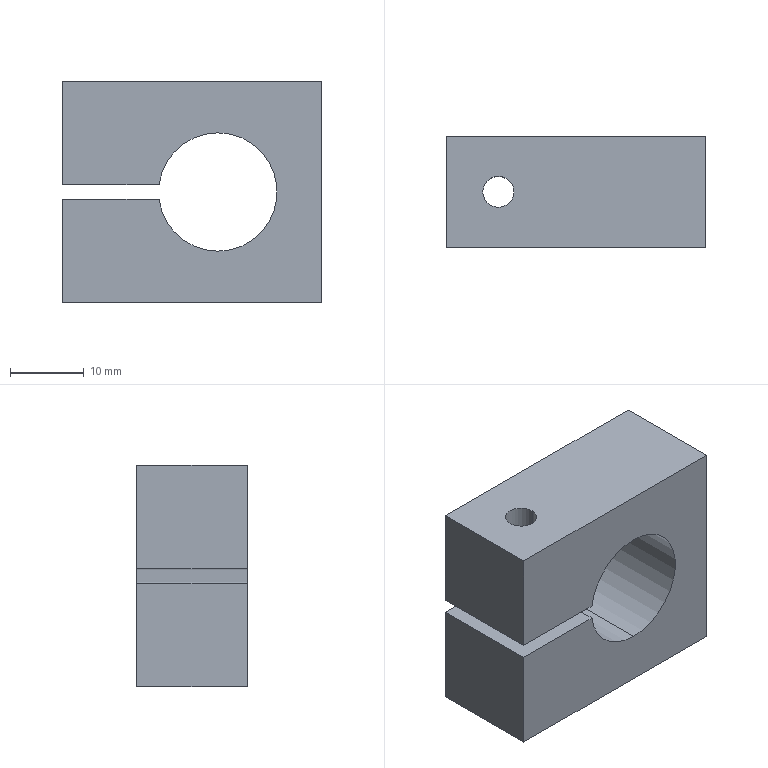Component | SolidWorks | PressingMechanism-11-5 | 1 solid | 19 faces | box 35 x 15 x 30 mm | volume 11521 mm3 | plane 10 | cylinder 9 | commonest cylinder face diameters 16 x3 10 x2 5.5 x2 4.2 x2
build123d program:
from build123d import *

# Parameters (mm, degrees)
SKETCH1_W                                           = 35
SKETCH1_H                                           = 30
EXTRUDE1_DEPTH                                      = 7.5
SKETCH2_R                                           = 8
EXTRUDE2_DEPTH                                      = 28.5
SKETCH3_W                                           = 21
SKETCH3_H                                           = 2
CUT_EXTRUDE_THIN2_DEPTH                             = 28.5
SKETCH4_W                                           = 2.1
SKETCH4_H                                           = 14
CBORE_FOR_M5_HEX_SOCKET_HEAD_CAP_SCREW1_D           = 5.5
CBORE_FOR_M5_HEX_SOCKET_HEAD_CAP_SCREW1_DEPTH       = 14
CBORE_FOR_M5_HEX_SOCKET_HEAD_CAP_SCREW1_CBORE_D     = 10
CBORE_FOR_M5_HEX_SOCKET_HEAD_CAP_SCREW1_CBORE_DEPTH = 5.4


with BuildPart() as part:
    # Sketch1 → Extrude1 (new, symmetric)
    with BuildSketch(Plane(origin=(0, 0, 0), x_dir=(1, 0, 0), z_dir=(0, 1, 0))):
        Rectangle(SKETCH1_W, SKETCH1_H)
    extrude(amount=EXTRUDE1_DEPTH, both=True)

    # Sketch2 → Extrude2 (cut, through all)
    with BuildSketch(Plane(origin=(0, 7.5, 0), x_dir=(1, 0, 0), z_dir=(0, 1, 0))):
        with Locations(Location((-3.5, 0, 0), (0, 0, 270))):
            Circle(SKETCH2_R)
    extrude(amount=-EXTRUDE2_DEPTH, mode=Mode.SUBTRACT)

    # Sketch3 → Cut-Extrude-Thin2 (cut, through all)
    with BuildSketch(Plane(origin=(0, 7.5, 0), x_dir=(1, 0, 0), z_dir=(0, 1, 0))):
        with Locations((7, 0)):
            Rectangle(SKETCH3_W, SKETCH3_H)
    extrude(amount=-CUT_EXTRUDE_THIN2_DEPTH, mode=Mode.SUBTRACT)

    # Sketch4 → M5 Tapped Hole1 (revolve, cut)
    with BuildSketch(Plane(origin=(10.5, 0, -1), x_dir=(0, -1, 0), z_dir=(1, 0, 0))):
        with Locations((1.05, 7)):
            Rectangle(SKETCH4_W, SKETCH4_H)
    revolve(axis=Axis((10.5, 0, 5.35), (0, 0, -1)), mode=Mode.SUBTRACT)

    # CBORE for M5 Hex Socket Head Cap Screw1
    with Locations(Plane.XY.offset(15)):
        with Locations((10.5, 0)):
            CounterBoreHole(CBORE_FOR_M5_HEX_SOCKET_HEAD_CAP_SCREW1_D / 2, CBORE_FOR_M5_HEX_SOCKET_HEAD_CAP_SCREW1_CBORE_D / 2, CBORE_FOR_M5_HEX_SOCKET_HEAD_CAP_SCREW1_CBORE_DEPTH, depth=CBORE_FOR_M5_HEX_SOCKET_HEAD_CAP_SCREW1_DEPTH)


solid = part.part

# Placed as in the assembly
solid = solid.moved(Location((-163.5, -77.889, 205), (-180, 0, 180)))
STEP:
#1=COLOUR_RGB('',0.7922,0.8196,0.9333);
#2=FILL_AREA_STYLE_COLOUR('',#1);
#3=FILL_AREA_STYLE('',(#2));
#4=SURFACE_STYLE_FILL_AREA(#3);
#5=SURFACE_SIDE_STYLE('',(#4));
#6=SURFACE_STYLE_USAGE(.BOTH.,#5);
#7=PRESENTATION_STYLE_ASSIGNMENT((#6));
#8=CARTESIAN_POINT('',(-6.654,-3.066,7.693));
#9=VERTEX_POINT('',#8);
#10=CARTESIAN_POINT('',(-7.047,-3.066,7.693));
#11=VERTEX_POINT('',#10);
#12=CARTESIAN_POINT('',(-6.85,-3.066,7.693));
#13=DIRECTION('',(0.,0.,-1.));
#14=DIRECTION('',(-1.,0.,0.));
#15=AXIS2_PLACEMENT_3D('',#12,#13,#14);
#16=CIRCLE('',#15,0.1969);
#17=EDGE_CURVE('',#9,#11,#16,.T.);
#18=ORIENTED_EDGE('',*,*,#17,.F.);
#19=CARTESIAN_POINT('',(-6.654,-3.066,7.48));
#20=VERTEX_POINT('',#19);
#21=CARTESIAN_POINT('',(-6.654,-3.066,7.48));
#22=DIRECTION('',(0.,0.,-1.));
#23=VECTOR('',#22,39.37);
#24=LINE('',#21,#23);
#25=EDGE_CURVE('',#9,#20,#24,.T.);
#26=ORIENTED_EDGE('',*,*,#25,.T.);
#27=CARTESIAN_POINT('',(-7.047,-3.066,7.48));
#28=VERTEX_POINT('',#27);
#29=CARTESIAN_POINT('',(-6.85,-3.066,7.48));
#30=DIRECTION('',(0.,0.,-1.));
#31=DIRECTION('',(-1.,0.,0.));
#32=AXIS2_PLACEMENT_3D('',#29,#30,#31);
#33=CIRCLE('',#32,0.1969);
#34=EDGE_CURVE('',#20,#28,#33,.T.);
#35=ORIENTED_EDGE('',*,*,#34,.T.);
#36=CARTESIAN_POINT('',(-7.047,-3.066,7.48));
#37=DIRECTION('',(0.,0.,-1.));
#38=VECTOR('',#37,39.37);
#39=LINE('',#36,#38);
#40=EDGE_CURVE('',#11,#28,#39,.T.);
#41=ORIENTED_EDGE('',*,*,#40,.F.);
#42=EDGE_LOOP('',(#18,#26,#35,#41));
#43=FACE_OUTER_BOUND('',#42,.T.);
#44=CARTESIAN_POINT('',(-6.85,-3.066,7.48));
#45=DIRECTION('',(0.,0.,-1.));
#46=DIRECTION('',(-1.,0.,0.));
#47=AXIS2_PLACEMENT_3D('',#44,#45,#46);
#48=CYLINDRICAL_SURFACE('',#47,0.1969);
#49=ADVANCED_FACE('',(#43),#48,.F.);
#50=CARTESIAN_POINT('',(-6.959,-3.066,8.031));
#51=VERTEX_POINT('',#50);
#52=CARTESIAN_POINT('',(-6.742,-3.066,8.031));
#53=VERTEX_POINT('',#52);
#54=CARTESIAN_POINT('',(-6.85,-3.066,8.031));
#55=DIRECTION('',(0.,0.,1.));
#56=DIRECTION('',(1.,0.,0.));
#57=AXIS2_PLACEMENT_3D('',#54,#55,#56);
#58=CIRCLE('',#57,0.1083);
#59=EDGE_CURVE('',#51,#53,#58,.T.);
#60=ORIENTED_EDGE('',*,*,#59,.T.);
#61=CARTESIAN_POINT('',(-6.742,-3.066,7.693));
#62=VERTEX_POINT('',#61);
#63=CARTESIAN_POINT('',(-6.742,-3.066,7.48));
#64=DIRECTION('',(0.,0.,-1.));
#65=VECTOR('',#64,39.37);
#66=LINE('',#63,#65);
#67=EDGE_CURVE('',#53,#62,#66,.T.);
#68=ORIENTED_EDGE('',*,*,#67,.T.);
#69=CARTESIAN_POINT('',(-6.959,-3.066,7.693));
#70=VERTEX_POINT('',#69);
#71=CARTESIAN_POINT('',(-6.85,-3.066,7.693));
#72=DIRECTION('',(0.,0.,-1.));
#73=DIRECTION('',(-1.,0.,0.));
#74=AXIS2_PLACEMENT_3D('',#71,#72,#73);
#75=CIRCLE('',#74,0.1083);
#76=EDGE_CURVE('',#62,#70,#75,.T.);
#77=ORIENTED_EDGE('',*,*,#76,.T.);
#78=CARTESIAN_POINT('',(-6.959,-3.066,7.48));
#79=DIRECTION('',(0.,0.,-1.));
#80=VECTOR('',#79,39.37);
#81=LINE('',#78,#80);
#82=EDGE_CURVE('',#51,#70,#81,.T.);
#83=ORIENTED_EDGE('',*,*,#82,.F.);
#84=EDGE_LOOP('',(#60,#68,#77,#83));
#85=FACE_OUTER_BOUND('',#84,.T.);
#86=CARTESIAN_POINT('',(-6.85,-3.066,7.48));
#87=DIRECTION('',(0.,0.,-1.));
#88=DIRECTION('',(-1.,0.,0.));
#89=AXIS2_PLACEMENT_3D('',#86,#87,#88);
#90=CYLINDRICAL_SURFACE('',#89,0.1083);
#91=ADVANCED_FACE('',(#85),#90,.F.);
#92=CARTESIAN_POINT('',(-6.768,-3.066,8.661));
#93=VERTEX_POINT('',#92);
#94=CARTESIAN_POINT('',(-6.933,-3.066,8.661));
#95=VERTEX_POINT('',#94);
#96=CARTESIAN_POINT('',(-6.85,-3.066,8.661));
#97=DIRECTION('',(0.,0.,-1.));
#98=DIRECTION('',(-1.,0.,0.));
#99=AXIS2_PLACEMENT_3D('',#96,#97,#98);
#100=CIRCLE('',#99,0.08268);
#101=EDGE_CURVE('',#93,#95,#100,.T.);
#102=ORIENTED_EDGE('',*,*,#101,.F.);
#103=CARTESIAN_POINT('',(-6.768,-3.066,8.11));
#104=VERTEX_POINT('',#103);
#105=CARTESIAN_POINT('',(-6.768,-3.066,8.11));
#106=DIRECTION('',(0.,0.,-1.));
#107=VECTOR('',#106,39.37);
#108=LINE('',#105,#107);
#109=EDGE_CURVE('',#93,#104,#108,.T.);
#110=ORIENTED_EDGE('',*,*,#109,.T.);
#111=CARTESIAN_POINT('',(-6.933,-3.066,8.11));
#112=VERTEX_POINT('',#111);
#113=CARTESIAN_POINT('',(-6.85,-3.066,8.11));
#114=DIRECTION('',(0.,0.,-1.));
#115=DIRECTION('',(-1.,0.,0.));
#116=AXIS2_PLACEMENT_3D('',#113,#114,#115);
#117=CIRCLE('',#116,0.08268);
#118=EDGE_CURVE('',#104,#112,#117,.T.);
#119=ORIENTED_EDGE('',*,*,#118,.T.);
#120=CARTESIAN_POINT('',(-6.933,-3.066,8.11));
#121=DIRECTION('',(0.,0.,-1.));
#122=VECTOR('',#121,39.37);
#123=LINE('',#120,#122);
#124=EDGE_CURVE('',#95,#112,#123,.T.);
#125=ORIENTED_EDGE('',*,*,#124,.F.);
#126=EDGE_LOOP('',(#102,#110,#119,#125));
#127=FACE_OUTER_BOUND('',#126,.T.);
#128=CARTESIAN_POINT('',(-6.85,-3.066,8.11));
#129=DIRECTION('',(0.,0.,-1.));
#130=DIRECTION('',(-1.,0.,0.));
#131=AXIS2_PLACEMENT_3D('',#128,#129,#130);
#132=CYLINDRICAL_SURFACE('',#131,0.08268);
#133=ADVANCED_FACE('',(#127),#132,.F.);
#134=CARTESIAN_POINT('',(-6.299,-3.362,8.386));
#135=VERTEX_POINT('',#134);
#136=CARTESIAN_POINT('',(-6.299,-3.362,7.756));
#137=VERTEX_POINT('',#136);
#138=CARTESIAN_POINT('',(-6.299,-3.362,8.071));
#139=DIRECTION('',(0.,1.,0.));
#140=DIRECTION('',(0.,0.,-1.));
#141=AXIS2_PLACEMENT_3D('',#138,#139,#140);
#142=CIRCLE('',#141,0.315);
#143=EDGE_CURVE('',#135,#137,#142,.T.);
#144=ORIENTED_EDGE('',*,*,#143,.F.);
#145=CARTESIAN_POINT('',(-6.299,-2.771,8.386));
#146=VERTEX_POINT('',#145);
#147=CARTESIAN_POINT('',(-6.299,-3.362,8.386));
#148=DIRECTION('',(0.,1.,0.));
#149=VECTOR('',#148,39.37);
#150=LINE('',#147,#149);
#151=EDGE_CURVE('',#135,#146,#150,.T.);
#152=ORIENTED_EDGE('',*,*,#151,.T.);
#153=CARTESIAN_POINT('',(-6.299,-2.771,7.756));
#154=VERTEX_POINT('',#153);
#155=CARTESIAN_POINT('',(-6.299,-2.771,8.071));
#156=DIRECTION('',(0.,1.,0.));
#157=DIRECTION('',(0.,0.,-1.));
#158=AXIS2_PLACEMENT_3D('',#155,#156,#157);
#159=CIRCLE('',#158,0.315);
#160=EDGE_CURVE('',#146,#154,#159,.T.);
#161=ORIENTED_EDGE('',*,*,#160,.T.);
#162=CARTESIAN_POINT('',(-6.299,-3.362,7.756));
#163=DIRECTION('',(0.,1.,0.));
#164=VECTOR('',#163,39.37);
#165=LINE('',#162,#164);
#166=EDGE_CURVE('',#137,#154,#165,.T.);
#167=ORIENTED_EDGE('',*,*,#166,.F.);
#168=EDGE_LOOP('',(#144,#152,#161,#167));
#169=FACE_OUTER_BOUND('',#168,.T.);
#170=CARTESIAN_POINT('',(-6.299,-3.362,8.071));
#171=DIRECTION('',(0.,1.,0.));
#172=DIRECTION('',(0.,0.,-1.));
#173=AXIS2_PLACEMENT_3D('',#170,#171,#172);
#174=CYLINDRICAL_SURFACE('',#173,0.315);
#175=ADVANCED_FACE('',(#169),#174,.F.);
#176=CARTESIAN_POINT('',(-6.612,-3.362,8.031));
#177=VERTEX_POINT('',#176);
#178=CARTESIAN_POINT('',(-6.299,-3.362,8.071));
#179=DIRECTION('',(0.,1.,0.));
#180=DIRECTION('',(0.,0.,-1.));
#181=AXIS2_PLACEMENT_3D('',#178,#179,#180);
#182=CIRCLE('',#181,0.315);
#183=EDGE_CURVE('',#137,#177,#182,.T.);
#184=ORIENTED_EDGE('',*,*,#183,.F.);
#185=ORIENTED_EDGE('',*,*,#166,.T.);
#186=CARTESIAN_POINT('',(-6.612,-2.771,8.031));
#187=VERTEX_POINT('',#186);
#188=CARTESIAN_POINT('',(-6.299,-2.771,8.071));
#189=DIRECTION('',(0.,1.,0.));
#190=DIRECTION('',(0.,0.,-1.));
#191=AXIS2_PLACEMENT_3D('',#188,#189,#190);
#192=CIRCLE('',#191,0.315);
#193=EDGE_CURVE('',#154,#187,#192,.T.);
#194=ORIENTED_EDGE('',*,*,#193,.T.);
#195=CARTESIAN_POINT('',(-6.612,-3.362,8.031));
#196=DIRECTION('',(0.,1.,0.));
#197=VECTOR('',#196,39.37);
#198=LINE('',#195,#197);
#199=EDGE_CURVE('',#177,#187,#198,.T.);
#200=ORIENTED_EDGE('',*,*,#199,.F.);
#201=EDGE_LOOP('',(#184,#185,#194,#200));
#202=FACE_OUTER_BOUND('',#201,.T.);
#203=CARTESIAN_POINT('',(-6.299,-3.362,8.071));
#204=DIRECTION('',(0.,1.,0.));
#205=DIRECTION('',(0.,0.,-1.));
#206=AXIS2_PLACEMENT_3D('',#203,#204,#205);
#207=CYLINDRICAL_SURFACE('',#206,0.315);
#208=ADVANCED_FACE('',(#202),#207,.F.);
#209=CARTESIAN_POINT('',(-7.126,-3.362,8.031));
#210=VERTEX_POINT('',#209);
#211=CARTESIAN_POINT('',(-7.126,-2.771,8.031));
#212=VERTEX_POINT('',#211);
#213=CARTESIAN_POINT('',(-7.126,-3.362,8.031));
#214=DIRECTION('',(0.,1.,0.));
#215=VECTOR('',#214,39.37);
#216=LINE('',#213,#215);
#217=EDGE_CURVE('',#210,#212,#216,.T.);
#218=ORIENTED_EDGE('',*,*,#217,.T.);
#219=CARTESIAN_POINT('',(-7.126,-2.771,7.48));
#220=VERTEX_POINT('',#219);
#221=CARTESIAN_POINT('',(-7.126,-2.771,8.661));
#222=DIRECTION('',(0.,0.,1.));
#223=VECTOR('',#222,39.37);
#224=LINE('',#221,#223);
#225=EDGE_CURVE('',#220,#212,#224,.T.);
#226=ORIENTED_EDGE('',*,*,#225,.F.);
#227=CARTESIAN_POINT('',(-7.126,-3.362,7.48));
#228=VERTEX_POINT('',#227);
#229=CARTESIAN_POINT('',(-7.126,-2.771,7.48));
#230=DIRECTION('',(0.,-1.,0.));
#231=VECTOR('',#230,39.37);
#232=LINE('',#229,#231);
#233=EDGE_CURVE('',#220,#228,#232,.T.);
#234=ORIENTED_EDGE('',*,*,#233,.T.);
#235=CARTESIAN_POINT('',(-7.126,-3.362,8.661));
#236=DIRECTION('',(0.,0.,1.));
#237=VECTOR('',#236,39.37);
#238=LINE('',#235,#237);
#239=EDGE_CURVE('',#228,#210,#238,.T.);
#240=ORIENTED_EDGE('',*,*,#239,.T.);
#241=EDGE_LOOP('',(#218,#226,#234,#240));
#242=FACE_OUTER_BOUND('',#241,.T.);
#243=CARTESIAN_POINT('',(-7.126,-2.771,8.661));
#244=DIRECTION('',(1.,0.,0.));
#245=DIRECTION('',(0.,0.,-1.));
#246=AXIS2_PLACEMENT_3D('',#243,#244,#245);
#247=PLANE('',#246);
#248=ADVANCED_FACE('',(#242),#247,.F.);
#249=CARTESIAN_POINT('',(-5.748,-3.362,8.661));
#250=VERTEX_POINT('',#249);
#251=CARTESIAN_POINT('',(-5.748,-3.362,7.48));
#252=VERTEX_POINT('',#251);
#253=CARTESIAN_POINT('',(-5.748,-3.362,8.661));
#254=DIRECTION('',(0.,0.,-1.));
#255=VECTOR('',#254,39.37);
#256=LINE('',#253,#255);
#257=EDGE_CURVE('',#250,#252,#256,.T.);
#258=ORIENTED_EDGE('',*,*,#257,.T.);
#259=CARTESIAN_POINT('',(-5.748,-2.771,7.48));
#260=VERTEX_POINT('',#259);
#261=CARTESIAN_POINT('',(-5.748,-2.771,7.48));
#262=DIRECTION('',(0.,-1.,0.));
#263=VECTOR('',#262,39.37);
#264=LINE('',#261,#263);
#265=EDGE_CURVE('',#260,#252,#264,.T.);
#266=ORIENTED_EDGE('',*,*,#265,.F.);
#267=CARTESIAN_POINT('',(-5.748,-2.771,8.661));
#268=VERTEX_POINT('',#267);
#269=CARTESIAN_POINT('',(-5.748,-2.771,8.661));
#270=DIRECTION('',(0.,0.,-1.));
#271=VECTOR('',#270,39.37);
#272=LINE('',#269,#271);
#273=EDGE_CURVE('',#268,#260,#272,.T.);
#274=ORIENTED_EDGE('',*,*,#273,.F.);
#275=CARTESIAN_POINT('',(-5.748,-2.771,8.661));
#276=DIRECTION('',(0.,-1.,0.));
#277=VECTOR('',#276,39.37);
#278=LINE('',#275,#277);
#279=EDGE_CURVE('',#268,#250,#278,.T.);
#280=ORIENTED_EDGE('',*,*,#279,.T.);
#281=EDGE_LOOP('',(#258,#266,#274,#280));
#282=FACE_OUTER_BOUND('',#281,.T.);
#283=CARTESIAN_POINT('',(-5.748,-2.771,8.661));
#284=DIRECTION('',(-1.,0.,0.));
#285=DIRECTION('',(0.,0.,1.));
#286=AXIS2_PLACEMENT_3D('',#283,#284,#285);
#287=PLANE('',#286);
#288=ADVANCED_FACE('',(#282),#287,.F.);
#289=CARTESIAN_POINT('',(-6.85,-3.066,7.48));
#290=DIRECTION('',(0.,0.,-1.));
#291=DIRECTION('',(-1.,0.,0.));
#292=AXIS2_PLACEMENT_3D('',#289,#290,#291);
#293=CIRCLE('',#292,0.1969);
#294=EDGE_CURVE('',#28,#20,#293,.T.);
#295=ORIENTED_EDGE('',*,*,#294,.F.);
#296=ORIENTED_EDGE('',*,*,#34,.F.);
#297=EDGE_LOOP('',(#295,#296));
#298=FACE_BOUND('',#297,.T.);
#299=CARTESIAN_POINT('',(-5.748,-3.362,7.48));
#300=DIRECTION('',(-1.,0.,0.));
#301=VECTOR('',#300,39.37);
#302=LINE('',#299,#301);
#303=EDGE_CURVE('',#252,#228,#302,.T.);
#304=ORIENTED_EDGE('',*,*,#303,.T.);
#305=ORIENTED_EDGE('',*,*,#233,.F.);
#306=CARTESIAN_POINT('',(-5.748,-2.771,7.48));
#307=DIRECTION('',(-1.,0.,0.));
#308=VECTOR('',#307,39.37);
#309=LINE('',#306,#308);
#310=EDGE_CURVE('',#260,#220,#309,.T.);
#311=ORIENTED_EDGE('',*,*,#310,.F.);
#312=ORIENTED_EDGE('',*,*,#265,.T.);
#313=EDGE_LOOP('',(#304,#305,#311,#312));
#314=FACE_OUTER_BOUND('',#313,.T.);
#315=CARTESIAN_POINT('',(-5.748,-2.771,7.48));
#316=DIRECTION('',(0.,0.,1.));
#317=DIRECTION('',(1.,0.,0.));
#318=AXIS2_PLACEMENT_3D('',#315,#316,#317);
#319=PLANE('',#318);
#320=ADVANCED_FACE('',(#298,#314),#319,.F.);
#321=CARTESIAN_POINT('',(-7.126,-2.771,8.11));
#322=VERTEX_POINT('',#321);
#323=CARTESIAN_POINT('',(-7.126,-2.771,8.661));
#324=VERTEX_POINT('',#323);
#325=CARTESIAN_POINT('',(-7.126,-2.771,8.661));
#326=DIRECTION('',(0.,0.,1.));
#327=VECTOR('',#326,39.37);
#328=LINE('',#325,#327);
#329=EDGE_CURVE('',#322,#324,#328,.T.);
#330=ORIENTED_EDGE('',*,*,#329,.F.);
#331=CARTESIAN_POINT('',(-7.126,-3.362,8.11));
#332=VERTEX_POINT('',#331);
#333=CARTESIAN_POINT('',(-7.126,-3.362,8.11));
#334=DIRECTION('',(0.,1.,0.));
#335=VECTOR('',#334,39.37);
#336=LINE('',#333,#335);
#337=EDGE_CURVE('',#332,#322,#336,.T.);
#338=ORIENTED_EDGE('',*,*,#337,.F.);
#339=CARTESIAN_POINT('',(-7.126,-3.362,8.661));
#340=VERTEX_POINT('',#339);
#341=CARTESIAN_POINT('',(-7.126,-3.362,8.661));
#342=DIRECTION('',(0.,0.,1.));
#343=VECTOR('',#342,39.37);
#344=LINE('',#341,#343);
#345=EDGE_CURVE('',#332,#340,#344,.T.);
#346=ORIENTED_EDGE('',*,*,#345,.T.);
#347=CARTESIAN_POINT('',(-7.126,-2.771,8.661));
#348=DIRECTION('',(0.,-1.,0.));
#349=VECTOR('',#348,39.37);
#350=LINE('',#347,#349);
#351=EDGE_CURVE('',#324,#340,#350,.T.);
#352=ORIENTED_EDGE('',*,*,#351,.F.);
#353=EDGE_LOOP('',(#330,#338,#346,#352));
#354=FACE_OUTER_BOUND('',#353,.T.);
#355=CARTESIAN_POINT('',(-7.126,-2.771,8.661));
#356=DIRECTION('',(1.,0.,0.));
#357=DIRECTION('',(0.,0.,-1.));
#358=AXIS2_PLACEMENT_3D('',#355,#356,#357);
#359=PLANE('',#358);
#360=ADVANCED_FACE('',(#354),#359,.F.);
#361=CARTESIAN_POINT('',(-6.85,-3.066,8.661));
#362=DIRECTION('',(0.,0.,-1.));
#363=DIRECTION('',(-1.,0.,0.));
#364=AXIS2_PLACEMENT_3D('',#361,#362,#363);
#365=CIRCLE('',#364,0.08268);
#366=EDGE_CURVE('',#95,#93,#365,.T.);
#367=ORIENTED_EDGE('',*,*,#366,.T.);
#368=ORIENTED_EDGE('',*,*,#101,.T.);
#369=EDGE_LOOP('',(#367,#368));
#370=FACE_BOUND('',#369,.T.);
#371=CARTESIAN_POINT('',(-5.748,-3.362,8.661));
#372=DIRECTION('',(1.,0.,0.));
#373=VECTOR('',#372,39.37);
#374=LINE('',#371,#373);
#375=EDGE_CURVE('',#340,#250,#374,.T.);
#376=ORIENTED_EDGE('',*,*,#375,.T.);
#377=ORIENTED_EDGE('',*,*,#279,.F.);
#378=CARTESIAN_POINT('',(-5.748,-2.771,8.661));
#379=DIRECTION('',(1.,0.,0.));
#380=VECTOR('',#379,39.37);
#381=LINE('',#378,#380);
#382=EDGE_CURVE('',#324,#268,#381,.T.);
#383=ORIENTED_EDGE('',*,*,#382,.F.);
#384=ORIENTED_EDGE('',*,*,#351,.T.);
#385=EDGE_LOOP('',(#376,#377,#383,#384));
#386=FACE_OUTER_BOUND('',#385,.T.);
#387=CARTESIAN_POINT('',(-5.748,-2.771,8.661));
#388=DIRECTION('',(0.,0.,-1.));
#389=DIRECTION('',(-1.,0.,0.));
#390=AXIS2_PLACEMENT_3D('',#387,#388,#389);
#391=PLANE('',#390);
#392=ADVANCED_FACE('',(#370,#386),#391,.F.);
#393=CARTESIAN_POINT('',(-6.612,-2.771,8.11));
#394=VERTEX_POINT('',#393);
#395=CARTESIAN_POINT('',(-7.126,-2.771,8.11));
#396=DIRECTION('',(1.,0.,0.));
#397=VECTOR('',#396,39.37);
#398=LINE('',#395,#397);
#399=EDGE_CURVE('',#322,#394,#398,.T.);
#400=ORIENTED_EDGE('',*,*,#399,.F.);
#401=ORIENTED_EDGE('',*,*,#329,.T.);
#402=ORIENTED_EDGE('',*,*,#382,.T.);
#403=ORIENTED_EDGE('',*,*,#273,.T.);
#404=ORIENTED_EDGE('',*,*,#310,.T.);
#405=ORIENTED_EDGE('',*,*,#225,.T.);
#406=CARTESIAN_POINT('',(-7.126,-2.771,8.031));
#407=DIRECTION('',(1.,0.,0.));
#408=VECTOR('',#407,39.37);
#409=LINE('',#406,#408);
#410=EDGE_CURVE('',#212,#187,#409,.T.);
#411=ORIENTED_EDGE('',*,*,#410,.T.);
#412=ORIENTED_EDGE('',*,*,#193,.F.);
#413=ORIENTED_EDGE('',*,*,#160,.F.);
#414=CARTESIAN_POINT('',(-6.299,-2.771,8.071));
#415=DIRECTION('',(0.,1.,0.));
#416=DIRECTION('',(0.,0.,-1.));
#417=AXIS2_PLACEMENT_3D('',#414,#415,#416);
#418=CIRCLE('',#417,0.315);
#419=EDGE_CURVE('',#394,#146,#418,.T.);
#420=ORIENTED_EDGE('',*,*,#419,.F.);
#421=EDGE_LOOP('',(#400,#401,#402,#403,#404,#405,#411,#412,#413,#420));
#422=FACE_OUTER_BOUND('',#421,.T.);
#423=CARTESIAN_POINT('',(-6.437,-2.771,8.071));
#424=DIRECTION('',(0.,1.,0.));
#425=DIRECTION('',(0.,0.,-1.));
#426=AXIS2_PLACEMENT_3D('',#423,#424,#425);
#427=PLANE('',#426);
#428=ADVANCED_FACE('',(#422),#427,.T.);
#429=ORIENTED_EDGE('',*,*,#345,.F.);
#430=CARTESIAN_POINT('',(-6.612,-3.362,8.11));
#431=VERTEX_POINT('',#430);
#432=CARTESIAN_POINT('',(-7.126,-3.362,8.11));
#433=DIRECTION('',(1.,0.,0.));
#434=VECTOR('',#433,39.37);
#435=LINE('',#432,#434);
#436=EDGE_CURVE('',#332,#431,#435,.T.);
#437=ORIENTED_EDGE('',*,*,#436,.T.);
#438=CARTESIAN_POINT('',(-6.299,-3.362,8.071));
#439=DIRECTION('',(0.,1.,0.));
#440=DIRECTION('',(0.,0.,-1.));
#441=AXIS2_PLACEMENT_3D('',#438,#439,#440);
#442=CIRCLE('',#441,0.315);
#443=EDGE_CURVE('',#431,#135,#442,.T.);
#444=ORIENTED_EDGE('',*,*,#443,.T.);
#445=ORIENTED_EDGE('',*,*,#143,.T.);
#446=ORIENTED_EDGE('',*,*,#183,.T.);
#447=CARTESIAN_POINT('',(-7.126,-3.362,8.031));
#448=DIRECTION('',(1.,0.,0.));
#449=VECTOR('',#448,39.37);
#450=LINE('',#447,#449);
#451=EDGE_CURVE('',#210,#177,#450,.T.);
#452=ORIENTED_EDGE('',*,*,#451,.F.);
#453=ORIENTED_EDGE('',*,*,#239,.F.);
#454=ORIENTED_EDGE('',*,*,#303,.F.);
#455=ORIENTED_EDGE('',*,*,#257,.F.);
#456=ORIENTED_EDGE('',*,*,#375,.F.);
#457=EDGE_LOOP('',(#429,#437,#444,#445,#446,#452,#453,#454,#455,#456));
#458=FACE_OUTER_BOUND('',#457,.T.);
#459=CARTESIAN_POINT('',(-6.437,-3.362,8.071));
#460=DIRECTION('',(0.,1.,0.));
#461=DIRECTION('',(0.,0.,-1.));
#462=AXIS2_PLACEMENT_3D('',#459,#460,#461);
#463=PLANE('',#462);
#464=ADVANCED_FACE('',(#458),#463,.F.);
#465=ORIENTED_EDGE('',*,*,#151,.F.);
#466=ORIENTED_EDGE('',*,*,#443,.F.);
#467=CARTESIAN_POINT('',(-6.612,-3.362,8.11));
#468=DIRECTION('',(0.,1.,0.));
#469=VECTOR('',#468,39.37);
#470=LINE('',#467,#469);
#471=EDGE_CURVE('',#431,#394,#470,.T.);
#472=ORIENTED_EDGE('',*,*,#471,.T.);
#473=ORIENTED_EDGE('',*,*,#419,.T.);
#474=EDGE_LOOP('',(#465,#466,#472,#473));
#475=FACE_OUTER_BOUND('',#474,.T.);
#476=CARTESIAN_POINT('',(-6.299,-3.362,8.071));
#477=DIRECTION('',(0.,1.,0.));
#478=DIRECTION('',(0.,0.,-1.));
#479=AXIS2_PLACEMENT_3D('',#476,#477,#478);
#480=CYLINDRICAL_SURFACE('',#479,0.315);
#481=ADVANCED_FACE('',(#475),#480,.F.);
#482=ORIENTED_EDGE('',*,*,#59,.F.);
#483=CARTESIAN_POINT('',(-6.85,-3.066,8.031));
#484=DIRECTION('',(0.,0.,1.));
#485=DIRECTION('',(1.,0.,0.));
#486=AXIS2_PLACEMENT_3D('',#483,#484,#485);
#487=CIRCLE('',#486,0.1083);
#488=EDGE_CURVE('',#53,#51,#487,.T.);
#489=ORIENTED_EDGE('',*,*,#488,.F.);
#490=EDGE_LOOP('',(#482,#489));
#491=FACE_BOUND('',#490,.T.);
#492=ORIENTED_EDGE('',*,*,#199,.T.);
#493=ORIENTED_EDGE('',*,*,#410,.F.);
#494=ORIENTED_EDGE('',*,*,#217,.F.);
#495=ORIENTED_EDGE('',*,*,#451,.T.);
#496=EDGE_LOOP('',(#492,#493,#494,#495));
#497=FACE_OUTER_BOUND('',#496,.T.);
#498=CARTESIAN_POINT('',(-7.126,-3.362,8.031));
#499=DIRECTION('',(0.,0.,1.));
#500=DIRECTION('',(1.,0.,0.));
#501=AXIS2_PLACEMENT_3D('',#498,#499,#500);
#502=PLANE('',#501);
#503=ADVANCED_FACE('',(#491,#497),#502,.T.);
#504=CARTESIAN_POINT('',(-6.85,-3.066,8.11));
#505=DIRECTION('',(0.,0.,-1.));
#506=DIRECTION('',(-1.,0.,0.));
#507=AXIS2_PLACEMENT_3D('',#504,#505,#506);
#508=CIRCLE('',#507,0.08268);
#509=EDGE_CURVE('',#112,#104,#508,.T.);
#510=ORIENTED_EDGE('',*,*,#509,.F.);
#511=ORIENTED_EDGE('',*,*,#118,.F.);
#512=EDGE_LOOP('',(#510,#511));
#513=FACE_BOUND('',#512,.T.);
#514=ORIENTED_EDGE('',*,*,#436,.F.);
#515=ORIENTED_EDGE('',*,*,#337,.T.);
#516=ORIENTED_EDGE('',*,*,#399,.T.);
#517=ORIENTED_EDGE('',*,*,#471,.F.);
#518=EDGE_LOOP('',(#514,#515,#516,#517));
#519=FACE_OUTER_BOUND('',#518,.T.);
#520=CARTESIAN_POINT('',(-7.126,-3.362,8.11));
#521=DIRECTION('',(0.,0.,1.));
#522=DIRECTION('',(1.,0.,0.));
#523=AXIS2_PLACEMENT_3D('',#520,#521,#522);
#524=PLANE('',#523);
#525=ADVANCED_FACE('',(#513,#519),#524,.F.);
#526=ORIENTED_EDGE('',*,*,#109,.F.);
#527=ORIENTED_EDGE('',*,*,#366,.F.);
#528=ORIENTED_EDGE('',*,*,#124,.T.);
#529=ORIENTED_EDGE('',*,*,#509,.T.);
#530=EDGE_LOOP('',(#526,#527,#528,#529));
#531=FACE_OUTER_BOUND('',#530,.T.);
#532=CARTESIAN_POINT('',(-6.85,-3.066,8.11));
#533=DIRECTION('',(0.,0.,-1.));
#534=DIRECTION('',(-1.,0.,0.));
#535=AXIS2_PLACEMENT_3D('',#532,#533,#534);
#536=CYLINDRICAL_SURFACE('',#535,0.08268);
#537=ADVANCED_FACE('',(#531),#536,.F.);
#538=ORIENTED_EDGE('',*,*,#67,.F.);
#539=ORIENTED_EDGE('',*,*,#488,.T.);
#540=ORIENTED_EDGE('',*,*,#82,.T.);
#541=CARTESIAN_POINT('',(-6.85,-3.066,7.693));
#542=DIRECTION('',(0.,0.,-1.));
#543=DIRECTION('',(-1.,0.,0.));
#544=AXIS2_PLACEMENT_3D('',#541,#542,#543);
#545=CIRCLE('',#544,0.1083);
#546=EDGE_CURVE('',#70,#62,#545,.T.);
#547=ORIENTED_EDGE('',*,*,#546,.T.);
#548=EDGE_LOOP('',(#538,#539,#540,#547));
#549=FACE_OUTER_BOUND('',#548,.T.);
#550=CARTESIAN_POINT('',(-6.85,-3.066,7.48));
#551=DIRECTION('',(0.,0.,-1.));
#552=DIRECTION('',(-1.,0.,0.));
#553=AXIS2_PLACEMENT_3D('',#550,#551,#552);
#554=CYLINDRICAL_SURFACE('',#553,0.1083);
#555=ADVANCED_FACE('',(#549),#554,.F.);
#556=ORIENTED_EDGE('',*,*,#546,.F.);
#557=ORIENTED_EDGE('',*,*,#76,.F.);
#558=EDGE_LOOP('',(#556,#557));
#559=FACE_BOUND('',#558,.T.);
#560=CARTESIAN_POINT('',(-6.85,-3.066,7.693));
#561=DIRECTION('',(0.,0.,-1.));
#562=DIRECTION('',(-1.,0.,0.));
#563=AXIS2_PLACEMENT_3D('',#560,#561,#562);
#564=CIRCLE('',#563,0.1969);
#565=EDGE_CURVE('',#11,#9,#564,.T.);
#566=ORIENTED_EDGE('',*,*,#565,.T.);
#567=ORIENTED_EDGE('',*,*,#17,.T.);
#568=EDGE_LOOP('',(#566,#567));
#569=FACE_OUTER_BOUND('',#568,.T.);
#570=CARTESIAN_POINT('',(-6.959,-3.066,7.693));
#571=DIRECTION('',(0.,0.,1.));
#572=DIRECTION('',(1.,0.,0.));
#573=AXIS2_PLACEMENT_3D('',#570,#571,#572);
#574=PLANE('',#573);
#575=ADVANCED_FACE('',(#559,#569),#574,.F.);
#576=ORIENTED_EDGE('',*,*,#25,.F.);
#577=ORIENTED_EDGE('',*,*,#565,.F.);
#578=ORIENTED_EDGE('',*,*,#40,.T.);
#579=ORIENTED_EDGE('',*,*,#294,.T.);
#580=EDGE_LOOP('',(#576,#577,#578,#579));
#581=FACE_OUTER_BOUND('',#580,.T.);
#582=CARTESIAN_POINT('',(-6.85,-3.066,7.48));
#583=DIRECTION('',(0.,0.,-1.));
#584=DIRECTION('',(-1.,0.,0.));
#585=AXIS2_PLACEMENT_3D('',#582,#583,#584);
#586=CYLINDRICAL_SURFACE('',#585,0.1969);
#587=ADVANCED_FACE('',(#581),#586,.F.);
#588=CLOSED_SHELL('',(#49,#91,#133,#175,#208,#248,#288,#320,#360,#392,#428,#464,#481,#503,#525,#537,#555,#575,#587));
#589=MANIFOLD_SOLID_BREP('',#588);
#590=STYLED_ITEM('',(#7),#589);
#591=PRESENTATION_LAYER_ASSIGNMENT('','',(#590));
#592=CARTESIAN_POINT('',(0.,0.,0.));
#593=DIRECTION('',(0.,0.,1.));
#594=DIRECTION('',(1.,0.,0.));
#595=AXIS2_PLACEMENT_3D('',#592,#593,#594);
#596=(LENGTH_UNIT()NAMED_UNIT(*)SI_UNIT($,.METRE.));
#597=LENGTH_MEASURE_WITH_UNIT(LENGTH_MEASURE(0.0254),#596);
#598=DIMENSIONAL_EXPONENTS(1.,0.,0.,0.,0.,0.,0.);
#599=(CONVERSION_BASED_UNIT('',#597)LENGTH_UNIT()NAMED_UNIT(#598));
#600=UNCERTAINTY_MEASURE_WITH_UNIT(LENGTH_MEASURE(0.00001),#599,'','');
#601=(NAMED_UNIT(*)PLANE_ANGLE_UNIT()SI_UNIT($,.RADIAN.));
#602=(NAMED_UNIT(*)SI_UNIT($,.STERADIAN.)SOLID_ANGLE_UNIT());
#603=(GEOMETRIC_REPRESENTATION_CONTEXT(3)GLOBAL_UNCERTAINTY_ASSIGNED_CONTEXT((#600))GLOBAL_UNIT_ASSIGNED_CONTEXT((#599,#601,#602))REPRESENTATION_CONTEXT('',''));
#604=ADVANCED_BREP_SHAPE_REPRESENTATION('',(#589,#595),#603);
#605=(LENGTH_UNIT()NAMED_UNIT(*)SI_UNIT($,.METRE.));
#606=LENGTH_MEASURE_WITH_UNIT(LENGTH_MEASURE(0.0254),#605);
#607=DIMENSIONAL_EXPONENTS(1.,0.,0.,0.,0.,0.,0.);
#608=(CONVERSION_BASED_UNIT('',#606)LENGTH_UNIT()NAMED_UNIT(#607));
#609=UNCERTAINTY_MEASURE_WITH_UNIT(LENGTH_MEASURE(0.00001),#608,'','');
#610=(NAMED_UNIT(*)PLANE_ANGLE_UNIT()SI_UNIT($,.RADIAN.));
#611=(NAMED_UNIT(*)SI_UNIT($,.STERADIAN.)SOLID_ANGLE_UNIT());
#612=(GEOMETRIC_REPRESENTATION_CONTEXT(3)GLOBAL_UNCERTAINTY_ASSIGNED_CONTEXT((#609))GLOBAL_UNIT_ASSIGNED_CONTEXT((#608,#610,#611))REPRESENTATION_CONTEXT('',''));
#613=MECHANICAL_DESIGN_GEOMETRIC_PRESENTATION_REPRESENTATION('',(#590),#612);